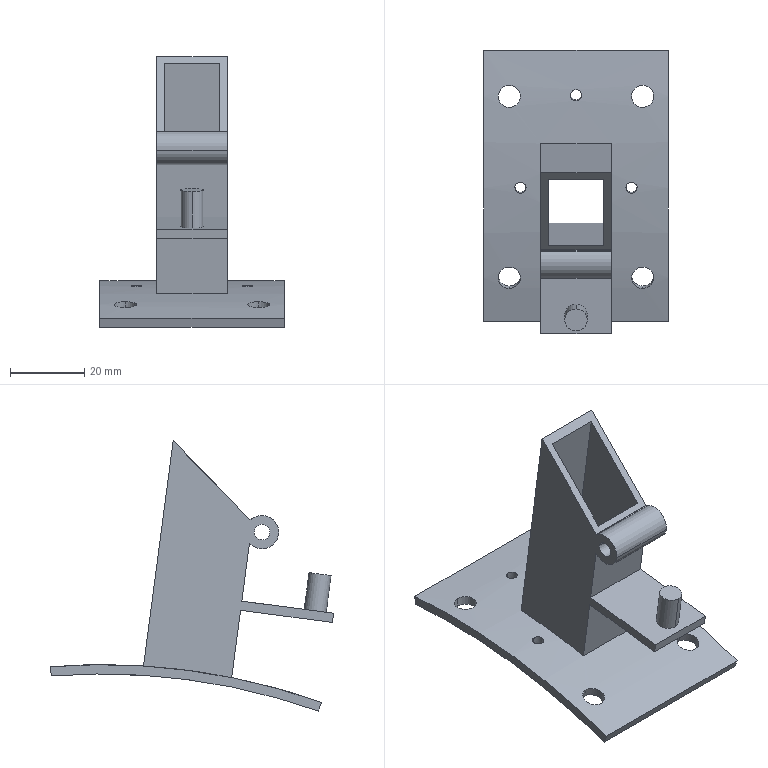Component | SolidWorks | SeedingAssemblyA-1_Duckbill-1 | 1 solid | 42 faces | box 49.9 x 76.44 x 72.97 mm | volume 18471 mm3 | cylinder 22 | plane 20 | commonest cylinder face diameters 6 x10 3 x6 4.2 x2 9 x2 355 x1 350 x1
build123d program:
from build123d import *

# Parameters (mm, degrees)
SKETCH1_2_R               = 177.5
SKETCH1_2_R_2             = 175
BOSS_EXTRUDE1_DEPTH       = 24.95
CUT_EXTRUDE1_2_DEPTH      = 256.935
CUT_EXTRUDE1_2_DEPTH_BACK = 256.935
SKETCH3_W                 = 15
SKETCH3_H                 = 20
CUT_EXTRUDE2_DEPTH        = 184.005
SKETCH4_W                 = 19
SKETCH4_H                 = 24
SKETCH4_W_2               = 15
SKETCH4_H_2               = 20
BOSS_EXTRUDE2_DEPTH       = 240
CUT_EXTRUDE3_DEPTH        = 246.252
CUT_EXTRUDE4_DEPTH        = 246.252
SKETCH9_R                 = 4.5
BOSS_EXTRUDE3_DEPTH       = 9.5
M5_TAPPED_HOLE1_D         = 4.2
SKETCH13_W                = 25
SKETCH13_H                = 2.5
BOSS_EXTRUDE4_DEPTH       = 19
SKETCH14_R                = 3
BOSS_EXTRUDE5_DEPTH       = 10
SKETCH15_R                = 1.5
CUT_EXTRUDE7_DEPTH        = 245.114
SKETCH16_R                = 1.5
CUT_EXTRUDE9_DEPTH        = 245.114
CUT_EXTRUDE1_DEPTH        = 10.5
CUT_EXTRUDE1_DEPTH_BACK   = 10.5


with BuildPart() as part:
    # Sketch1_2 → Boss-Extrude1 (new, symmetric)
    with BuildSketch(Plane(origin=(0, 0, 0), x_dir=(0, 0, -1), z_dir=(1, 0, 0))):
        Circle(SKETCH1_2_R)
        Circle(SKETCH1_2_R_2, mode=Mode.SUBTRACT)
    extrude(amount=BOSS_EXTRUDE1_DEPTH, both=True)

    # Sketch2 → Cut-Extrude1_2 (cut, two sides: drawn at the far end of the back side and taken through both)
    with BuildSketch(Plane(origin=(24.95, 0, 0), x_dir=(0, 0, -1), z_dir=(1, 0, 0)).offset(-CUT_EXTRUDE1_2_DEPTH_BACK)):
        Polygon((-210.056, 988.235), (-36.904, 173.621), (0, 0), (36.904, 173.621), (210.056, 988.235), (210.056, -677.391), (-210.056, -677.391), align=None)
    extrude(amount=CUT_EXTRUDE1_2_DEPTH + CUT_EXTRUDE1_2_DEPTH_BACK, mode=Mode.SUBTRACT)

    # Sketch3 → Cut-Extrude2 (cut, through all)
    with BuildSketch(Plane(origin=(0, 0, 0), x_dir=(1, 0, 0), z_dir=(0, 1, 0))):
        Rectangle(SKETCH3_W, SKETCH3_H)
    extrude(amount=CUT_EXTRUDE2_DEPTH, mode=Mode.SUBTRACT)

    # Sketch4 → Boss-Extrude2 (add)
    with BuildSketch(Plane(origin=(0, 0, 0), x_dir=(1, 0, 0), z_dir=(0, 1, 0))):
        Rectangle(SKETCH4_W, SKETCH4_H)
        Rectangle(SKETCH4_W_2, SKETCH4_H_2, mode=Mode.SUBTRACT)
    extrude(amount=BOSS_EXTRUDE2_DEPTH)

    # Sketch5 → Cut-Extrude3 (cut, through all)
    with BuildSketch(Plane.ZY.offset(9.5)):
        with BuildLine():
            Line((-12, 174.588), (-12, 0))
            Line((-12, 0), (12, 0))
            Line((12, 0), (12, 174.588))
            ThreePointArc((12, 174.588), (0, 175), (-12, 174.588))
        make_face()
    extrude(amount=-CUT_EXTRUDE3_DEPTH, mode=Mode.SUBTRACT)

    # Sketch6 → Cut-Extrude4 (cut, through all)
    with BuildSketch(Plane.ZY.offset(9.5)):
        Polygon((-12, 240), (12, 220), (12, 240), align=None)
    extrude(amount=-CUT_EXTRUDE4_DEPTH, mode=Mode.SUBTRACT)

    # Sketch8 → Cut-Revolve1 (revolve, cut)
    with BuildSketch(Plane(origin=(18, 0, 0), x_dir=(0, 0, -1), z_dir=(1, 0, 0))):
        Polygon((-24.94, 177.46), (-27.911, 177.042), (-26.1, 164.154), (-23.129, 164.572), align=None)
    cut_revolve1 = revolve(axis=Axis((18, 177.46, 24.94), (0, -0.9903, -0.1392)), mode=Mode.SUBTRACT)

    # Mirror1: Cut-Revolve1 across plane
    add(cut_revolve1.mirror(Plane.XY), mode=Mode.SUBTRACT)

    # Mirror2: Cut-Revolve1 across plane
    add(cut_revolve1.mirror(Plane(origin=(0, 0, 0), x_dir=(0, 0, 1), z_dir=(1, 0, 0))), mode=Mode.SUBTRACT)

    # Mirror2 copy 1 sketch → Mirror2 copy 1 (revolve, cut)
    with BuildSketch(Plane.ZY.offset(18)):
        Polygon((-24.94, 177.46), (-27.911, 177.042), (-26.1, 164.154), (-23.129, 164.572), align=None)
    revolve(axis=Axis((-18, 177.46, -24.94), (0, -0.9903, 0.1392)), mode=Mode.SUBTRACT)

    # Sketch9 → Boss-Extrude3 (add, symmetric)
    with BuildSketch(Plane(origin=(0, 0, 0), x_dir=(0, 0, -1), z_dir=(1, 0, 0))):
        with Locations((-15, 217.094)):
            Circle(SKETCH9_R)
    extrude(amount=BOSS_EXTRUDE3_DEPTH, both=True)

    # M5 Tapped Hole1 (through all)
    with Locations(Plane.ZY.offset(9.5)):
        with Locations((15, 217.094)):
            Hole(M5_TAPPED_HOLE1_D / 2)

    # Sketch13 → Boss-Extrude4 (add)
    with BuildSketch(Plane.ZY.offset(9.5)):
        with Locations((24.5, 196.667)):
            Rectangle(SKETCH13_W, SKETCH13_H)
    extrude(amount=-BOSS_EXTRUDE4_DEPTH)

    # Sketch14 → Boss-Extrude5 (add)
    with BuildSketch(Plane(origin=(0, 197.917, 0), x_dir=(1, 0, 0), z_dir=(0, 1, 0))):
        with Locations(Location((0, -32, 0), (0, 0, 270))):
            Circle(SKETCH14_R)
    extrude(amount=BOSS_EXTRUDE5_DEPTH)

    # Sketch15 → Cut-Extrude7 (cut, through all)
    with BuildSketch(Plane(origin=(0, 0, 0), x_dir=(1, 0, 0), z_dir=(0, 1, 0))):
        with Locations(Location((0, 25, 0), (0, 0, 90))):
            Circle(SKETCH15_R)
    extrude(amount=CUT_EXTRUDE7_DEPTH, mode=Mode.SUBTRACT)

    # Sketch16 → Cut-Extrude9 (cut, through all)
    with BuildSketch(Plane(origin=(0, 0, 0), x_dir=(1, 0, 0), z_dir=(0, 1, 0))):
        with Locations(Location((-15, 0, 0), (0, 0, 90))):
            Circle(SKETCH16_R)
        with Locations(Location((15, 0, 0), (0, 0, 90))):
            Circle(SKETCH16_R)
    extrude(amount=CUT_EXTRUDE9_DEPTH, mode=Mode.SUBTRACT)

    # Sketch1 → Cut-Extrude1 (cut, two sides: drawn at the far end of the back side and taken through both)
    with BuildSketch(Plane(origin=(0, 0, 0), x_dir=(0, 0, -1), z_dir=(1, 0, 0)).offset(-CUT_EXTRUDE1_DEPTH_BACK)):
        Polygon((15, 240.773), (-11.269, 220.033), (-11.774, 220.581), (-13.695, 222.885), (15, 247), align=None)
    extrude(amount=CUT_EXTRUDE1_DEPTH + CUT_EXTRUDE1_DEPTH_BACK, mode=Mode.SUBTRACT)


solid = part.part

# Placed as in the assembly
solid = solid.moved(Location((90.731, -105.002, -252.184), (97.503, 0, 0)))